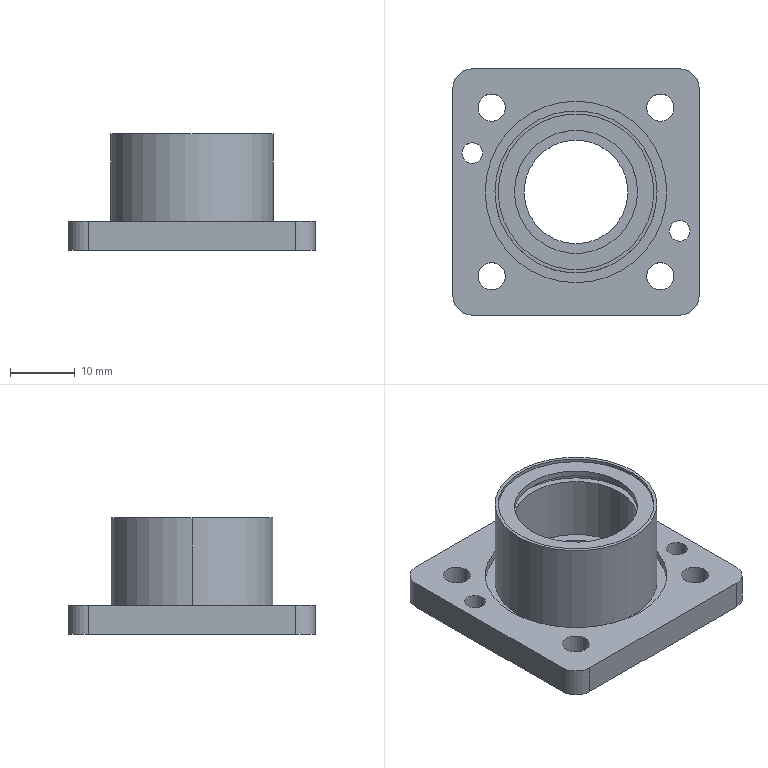CAM job | Mastercam | mm | 4 operations | part box 38 x 38 x 17.95
1. Contour (Ramp) | 8 - 8 平铣刀
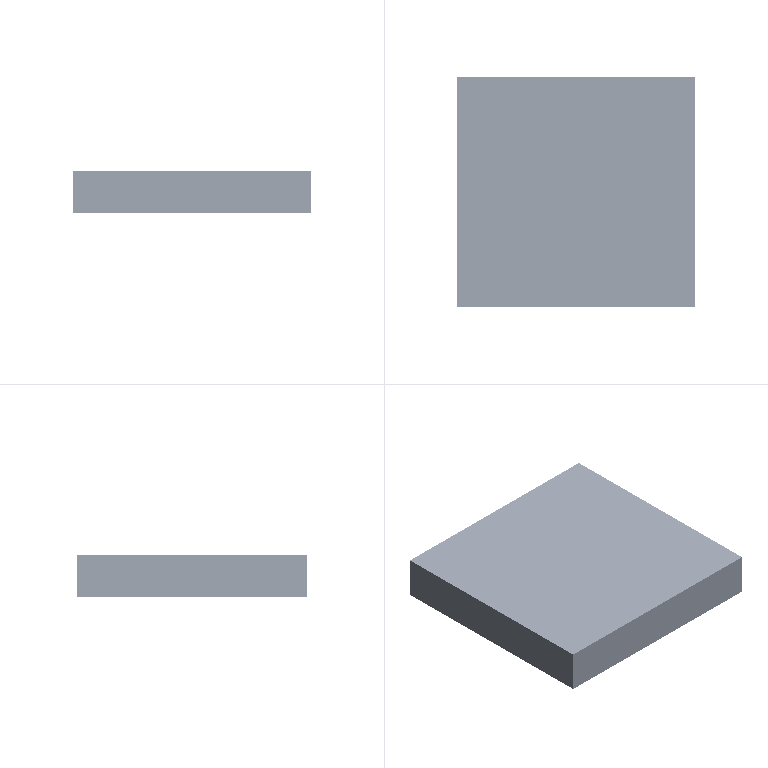2. Contour (2D) | 8 - 8 平铣刀
3. Drill/Counterbore | 7 - 4 倒角刀
4. Contour (2D chamfer) | 7 - 4 倒角刀